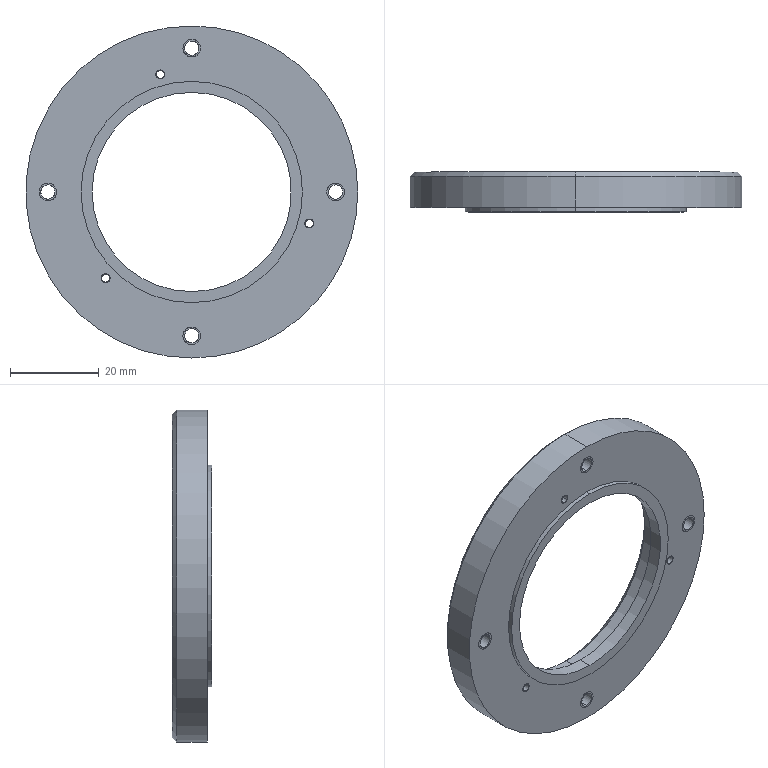CAM job | Mastercam | mm | 1 operations | part box 75 x 9 x 75
1. Drill/Counterbore | 7 - 4 倒角刀